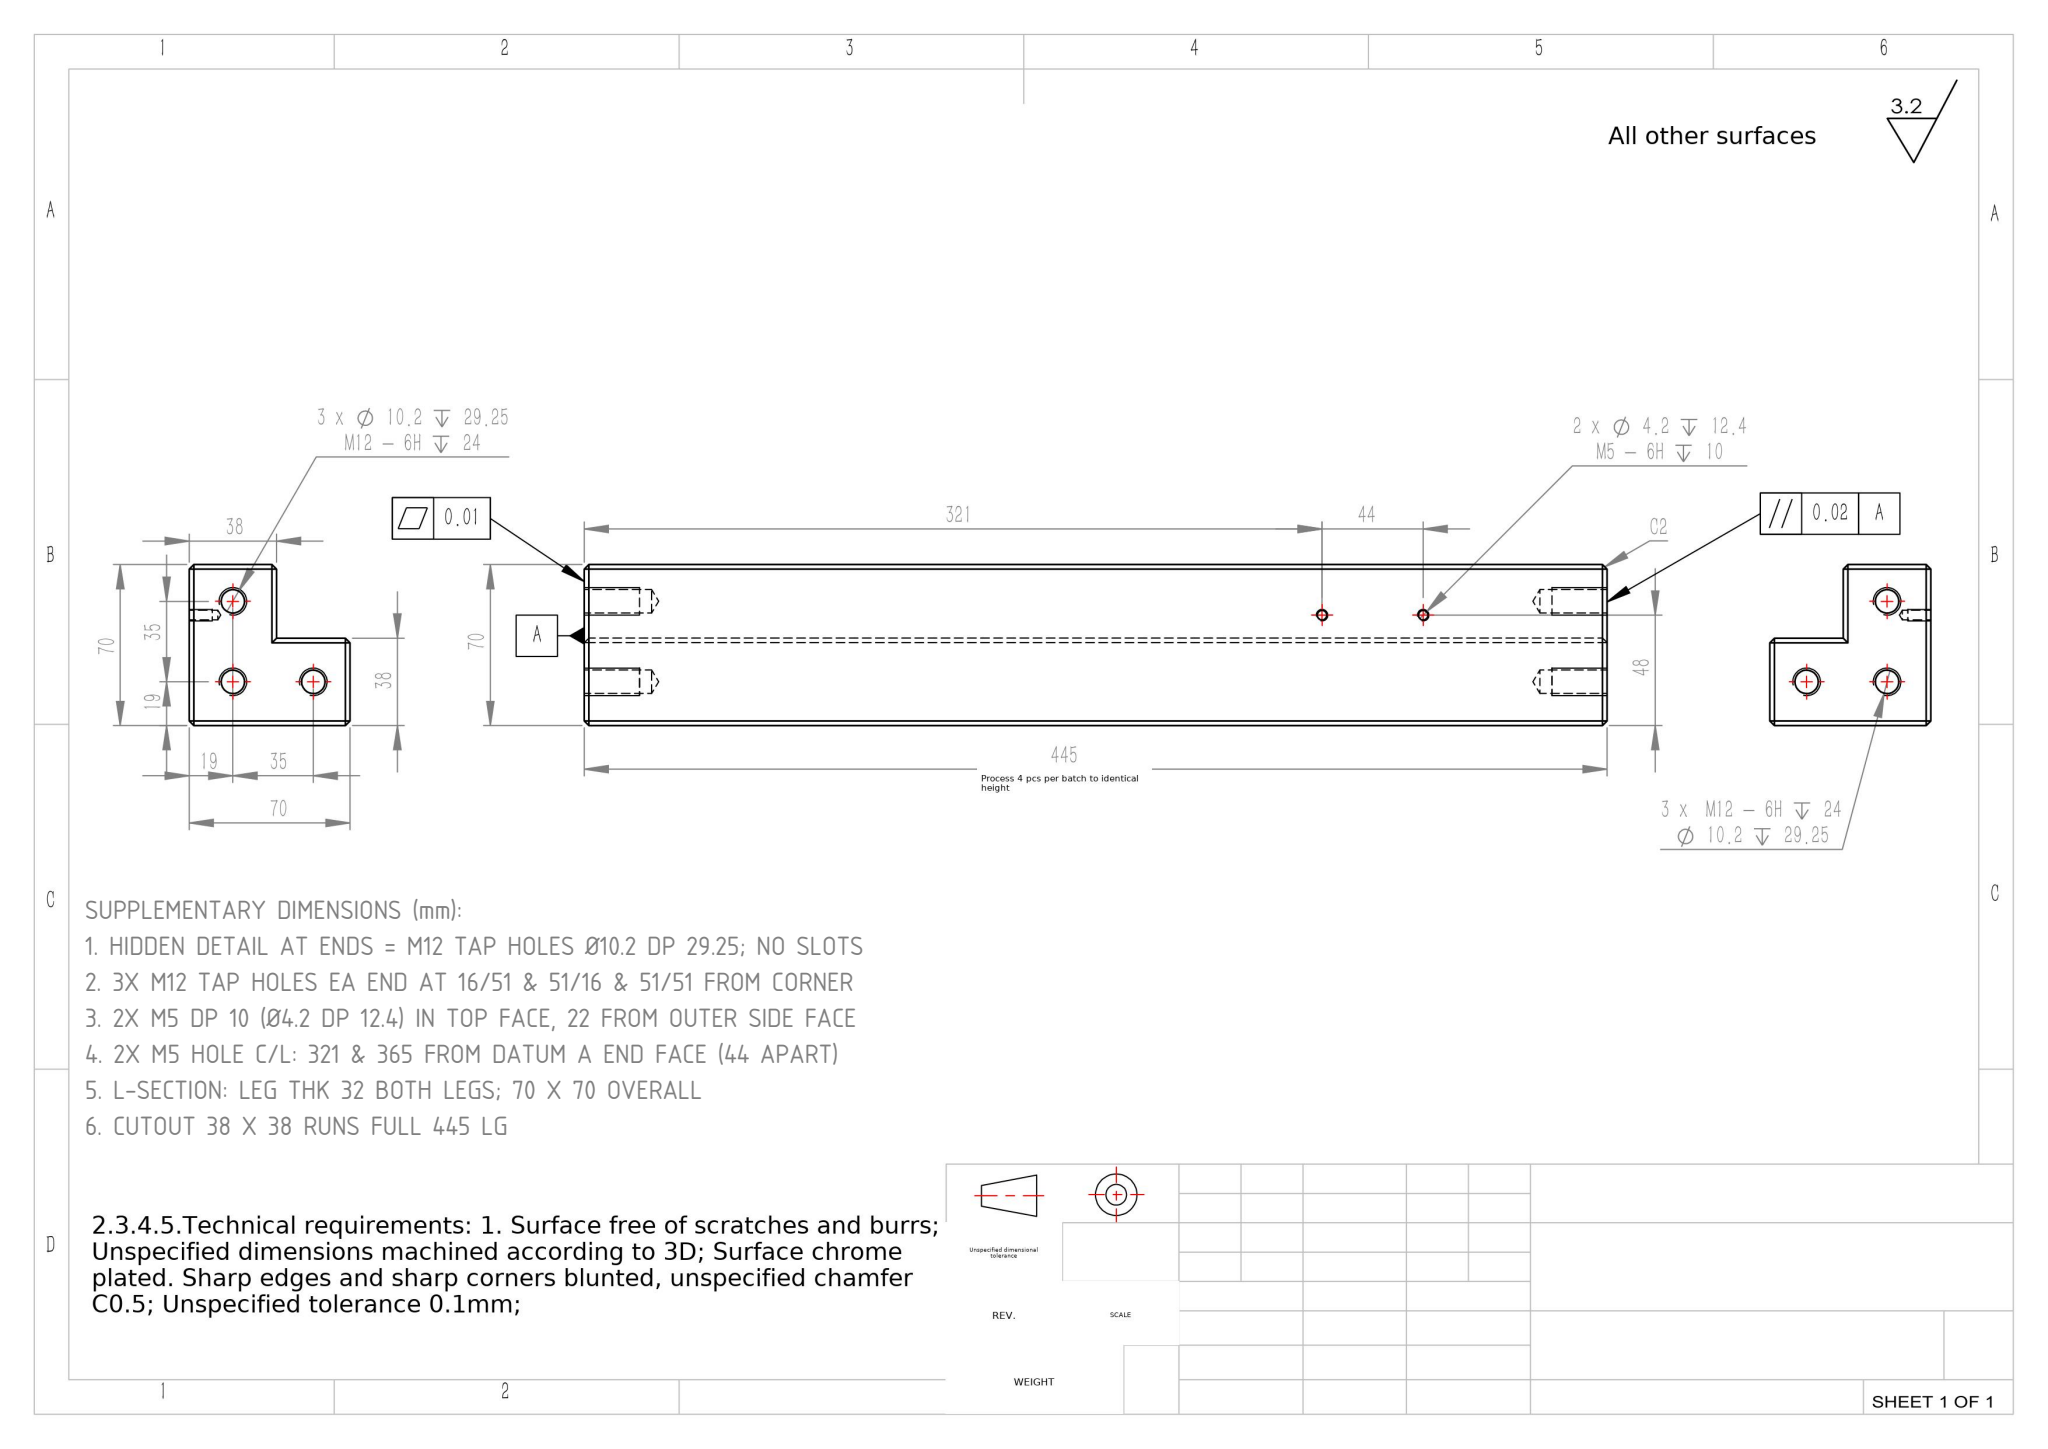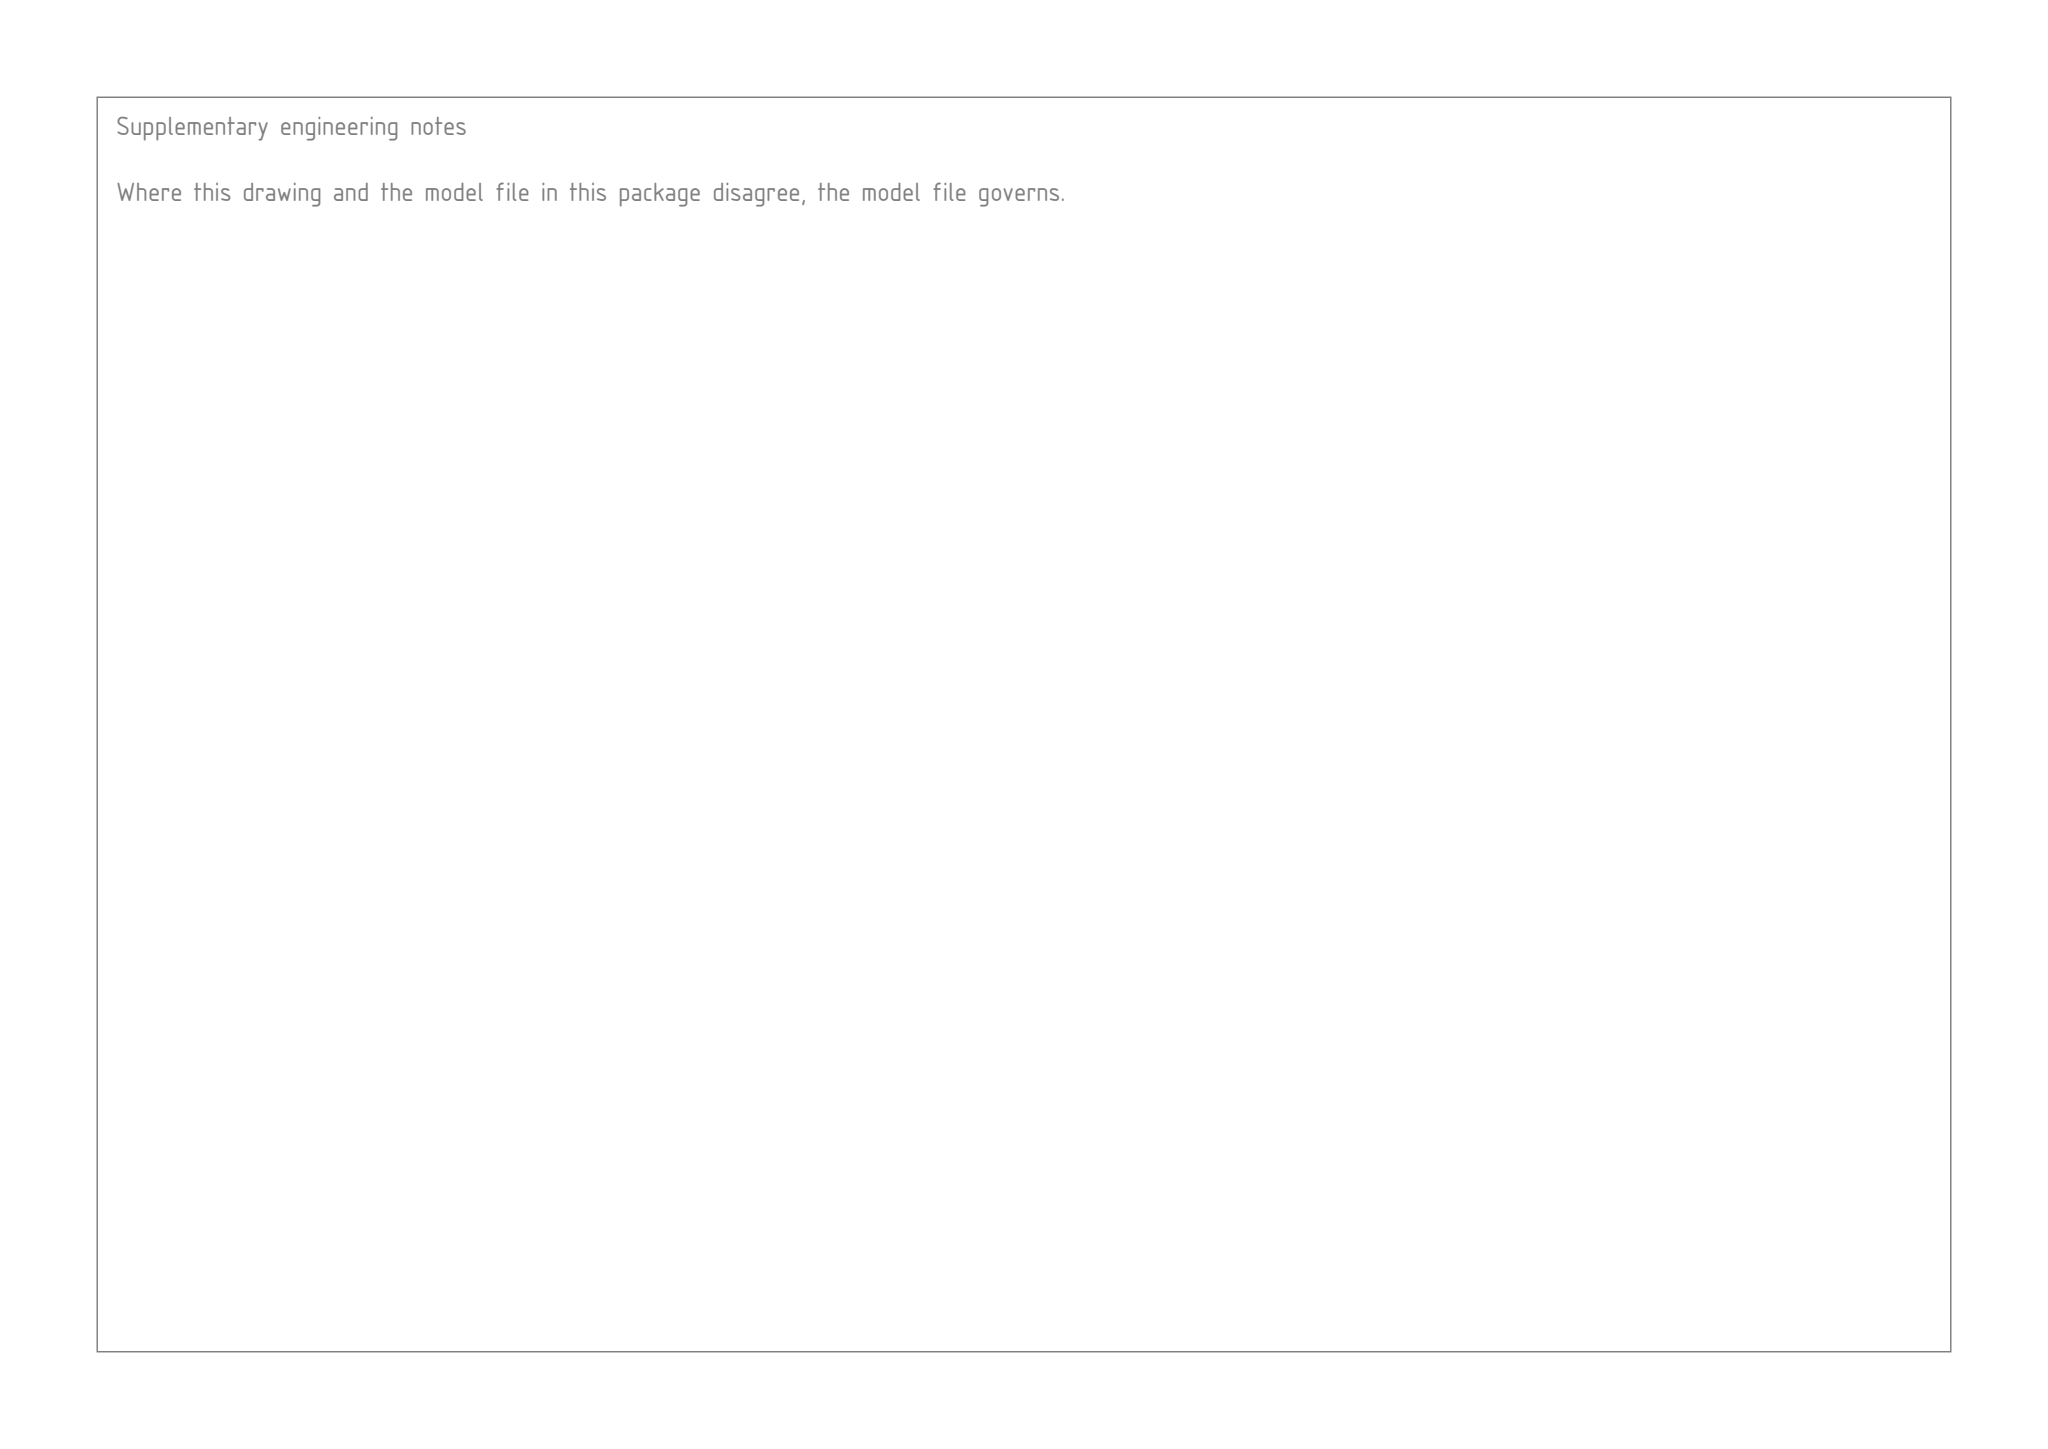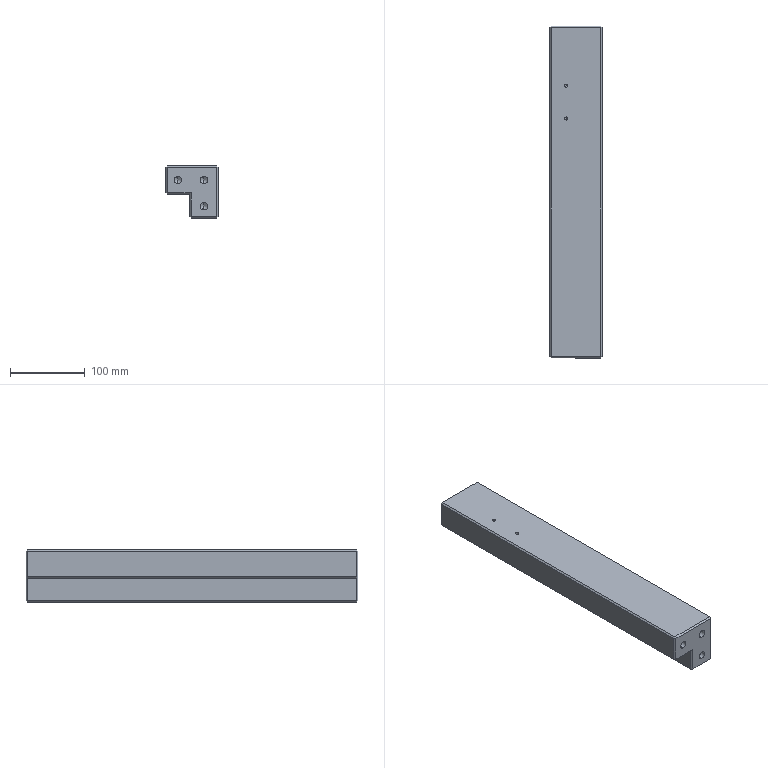Part | SolidWorks | mm | 1 solid | 67 faces | box 70 x 445 x 70 mm | volume 1704101 mm3 | plane 35 | cylinder 16 | cone 16 | commonest cylinder face diameters 10.2 x12 4.2 x4
build123d program:
from build123d import *

# Parameters (mm, degrees)
SKETCH1_W              = 70
SKETCH1_H              = 445
BOSS_EXTRUDE1_DEPTH    = 35
SKETCH2_W              = 32
SKETCH2_H              = 32
CUT_EXTRUDE1_DEPTH     = 448.744
M12_TAPPED_HOLE1_D     = 10.2
M12_TAPPED_HOLE1_DEPTH = 29.25
M12_TAPPED_HOLE1_TIP   = 3.064
M12_TAPPED_HOLE2_D     = 10.2
M12_TAPPED_HOLE2_DEPTH = 29.25
M12_TAPPED_HOLE2_TIP   = 3.064
CHAMFER1_SIZE          = 2
M5_TAPPED_HOLE1_D      = 4.2
M5_TAPPED_HOLE1_DEPTH  = 12.4
M5_TAPPED_HOLE1_TIP    = 1.262


with BuildPart() as part:
    # Sketch1 → Boss-Extrude1 (new, symmetric)
    with BuildSketch(Plane.XY):
        Rectangle(SKETCH1_W, SKETCH1_H)
    extrude(amount=BOSS_EXTRUDE1_DEPTH, both=True)

    # Sketch2 → Cut-Extrude1 (cut, through all)
    with BuildSketch(Plane(origin=(0, 222.5, 0), x_dir=(1, 0, 0), z_dir=(0, 1, 0))):
        with Locations((-19, 19)):
            Rectangle(SKETCH2_W, SKETCH2_H)
    extrude(amount=-CUT_EXTRUDE1_DEPTH, mode=Mode.SUBTRACT)

    # M12 Tapped Hole1
    with Locations(Plane(origin=(0, 222.5, 0), x_dir=(1, 0, 0), z_dir=(0, 1, 0))):
        with Locations((16, 19), (16, -16), (-19, -16)):
            Hole(M12_TAPPED_HOLE1_D / 2, depth=M12_TAPPED_HOLE1_DEPTH)
            with Locations((0, 0, -(M12_TAPPED_HOLE1_DEPTH + M12_TAPPED_HOLE1_TIP / 2))):  # 118° drill point
                Cone(0, M12_TAPPED_HOLE1_D / 2, M12_TAPPED_HOLE1_TIP, mode=Mode.SUBTRACT)

    # M12 Tapped Hole2
    with Locations(Plane(origin=(0, -222.5, 0), x_dir=(-1, 0, 0), z_dir=(0, -1, 0))):
        with Locations((19, -16), (-16, -16), (-16, 19)):
            Hole(M12_TAPPED_HOLE2_D / 2, depth=M12_TAPPED_HOLE2_DEPTH)
            with Locations((0, 0, -(M12_TAPPED_HOLE2_DEPTH + M12_TAPPED_HOLE2_TIP / 2))):  # 118° drill point
                Cone(0, M12_TAPPED_HOLE2_D / 2, M12_TAPPED_HOLE2_TIP, mode=Mode.SUBTRACT)

    # Chamfer1
    chamfer1_edges = [part.edges().sort_by_distance(p)[0] for p in [
        (-35, 0, 35),
        (16, -222.5, -35),
        (0, -222.5, 35),
        (-35, 0, -3),
        (-3, -222.5, -19),
        (-3, 0, -35),
        (-19, -222.5, -3),
        (-19, 222.5, -3),
        (-3, 222.5, -19),
        (35, 0, 35),
        (16, 222.5, -35),
        (35, 0, -35),
        (35, -222.5, 0),
        (-35, -222.5, 16),
        (-35, 222.5, 16),
        (35, 222.5, 0),
        (0, 222.5, 35),
    ]]
    chamfer(chamfer1_edges, length=CHAMFER1_SIZE)

    # M5 Tapped Hole1
    with Locations(Plane.XY.offset(35)):
        with Locations((-13, 142.5), (-13, 98.5)):
            Hole(M5_TAPPED_HOLE1_D / 2, depth=M5_TAPPED_HOLE1_DEPTH)
            with Locations((0, 0, -(M5_TAPPED_HOLE1_DEPTH + M5_TAPPED_HOLE1_TIP / 2))):  # 118° drill point
                Cone(0, M5_TAPPED_HOLE1_D / 2, M5_TAPPED_HOLE1_TIP, mode=Mode.SUBTRACT)


solid = part.part